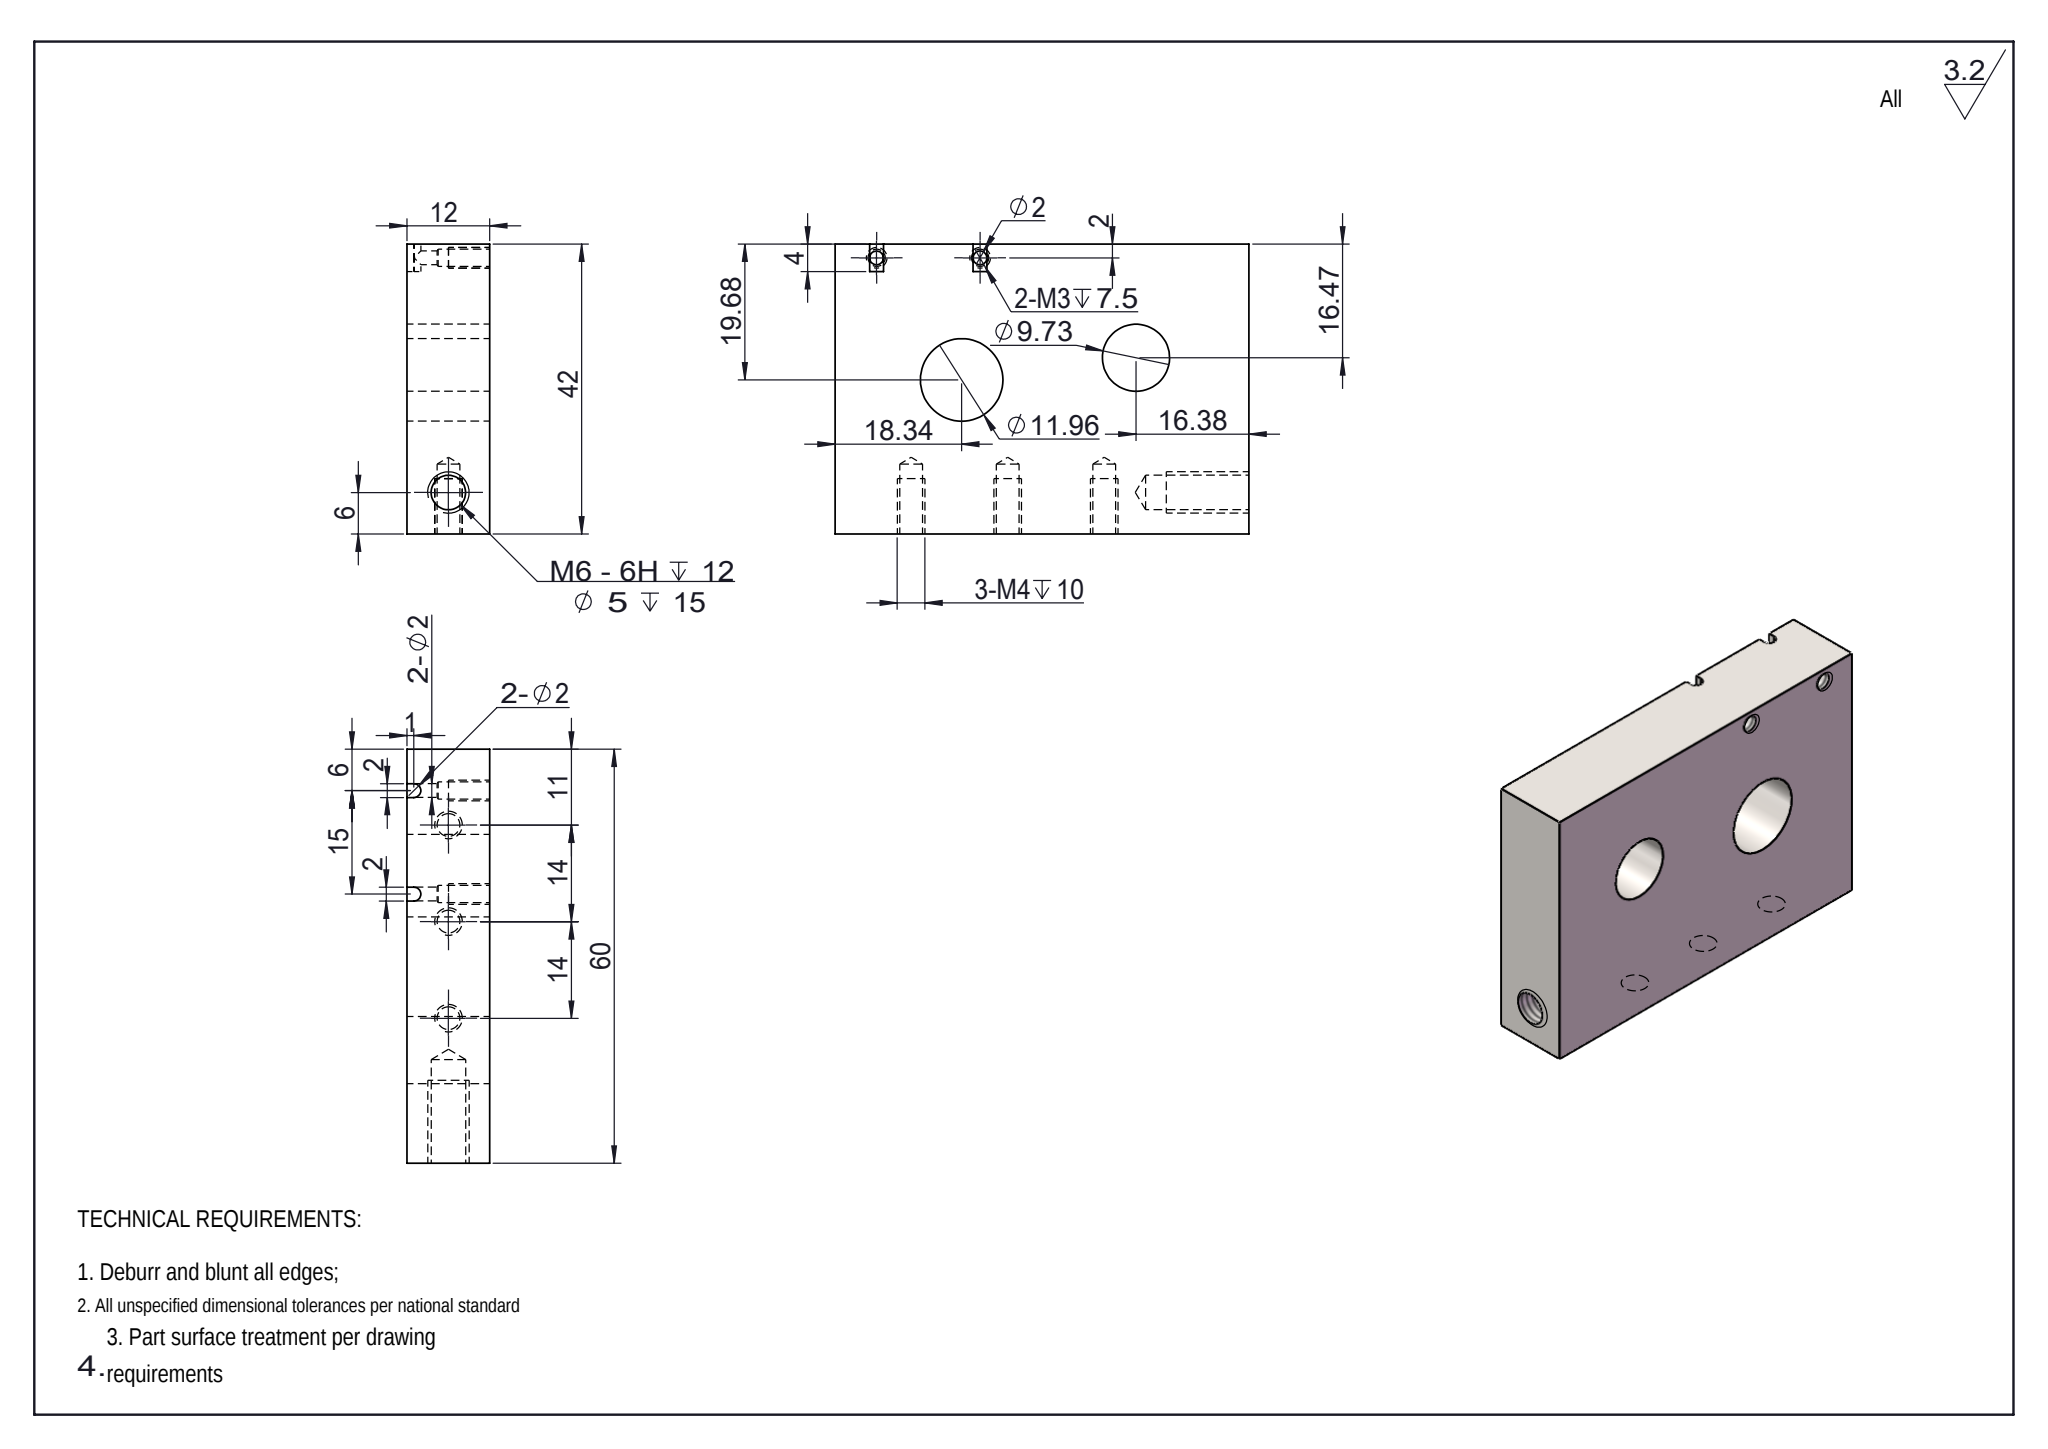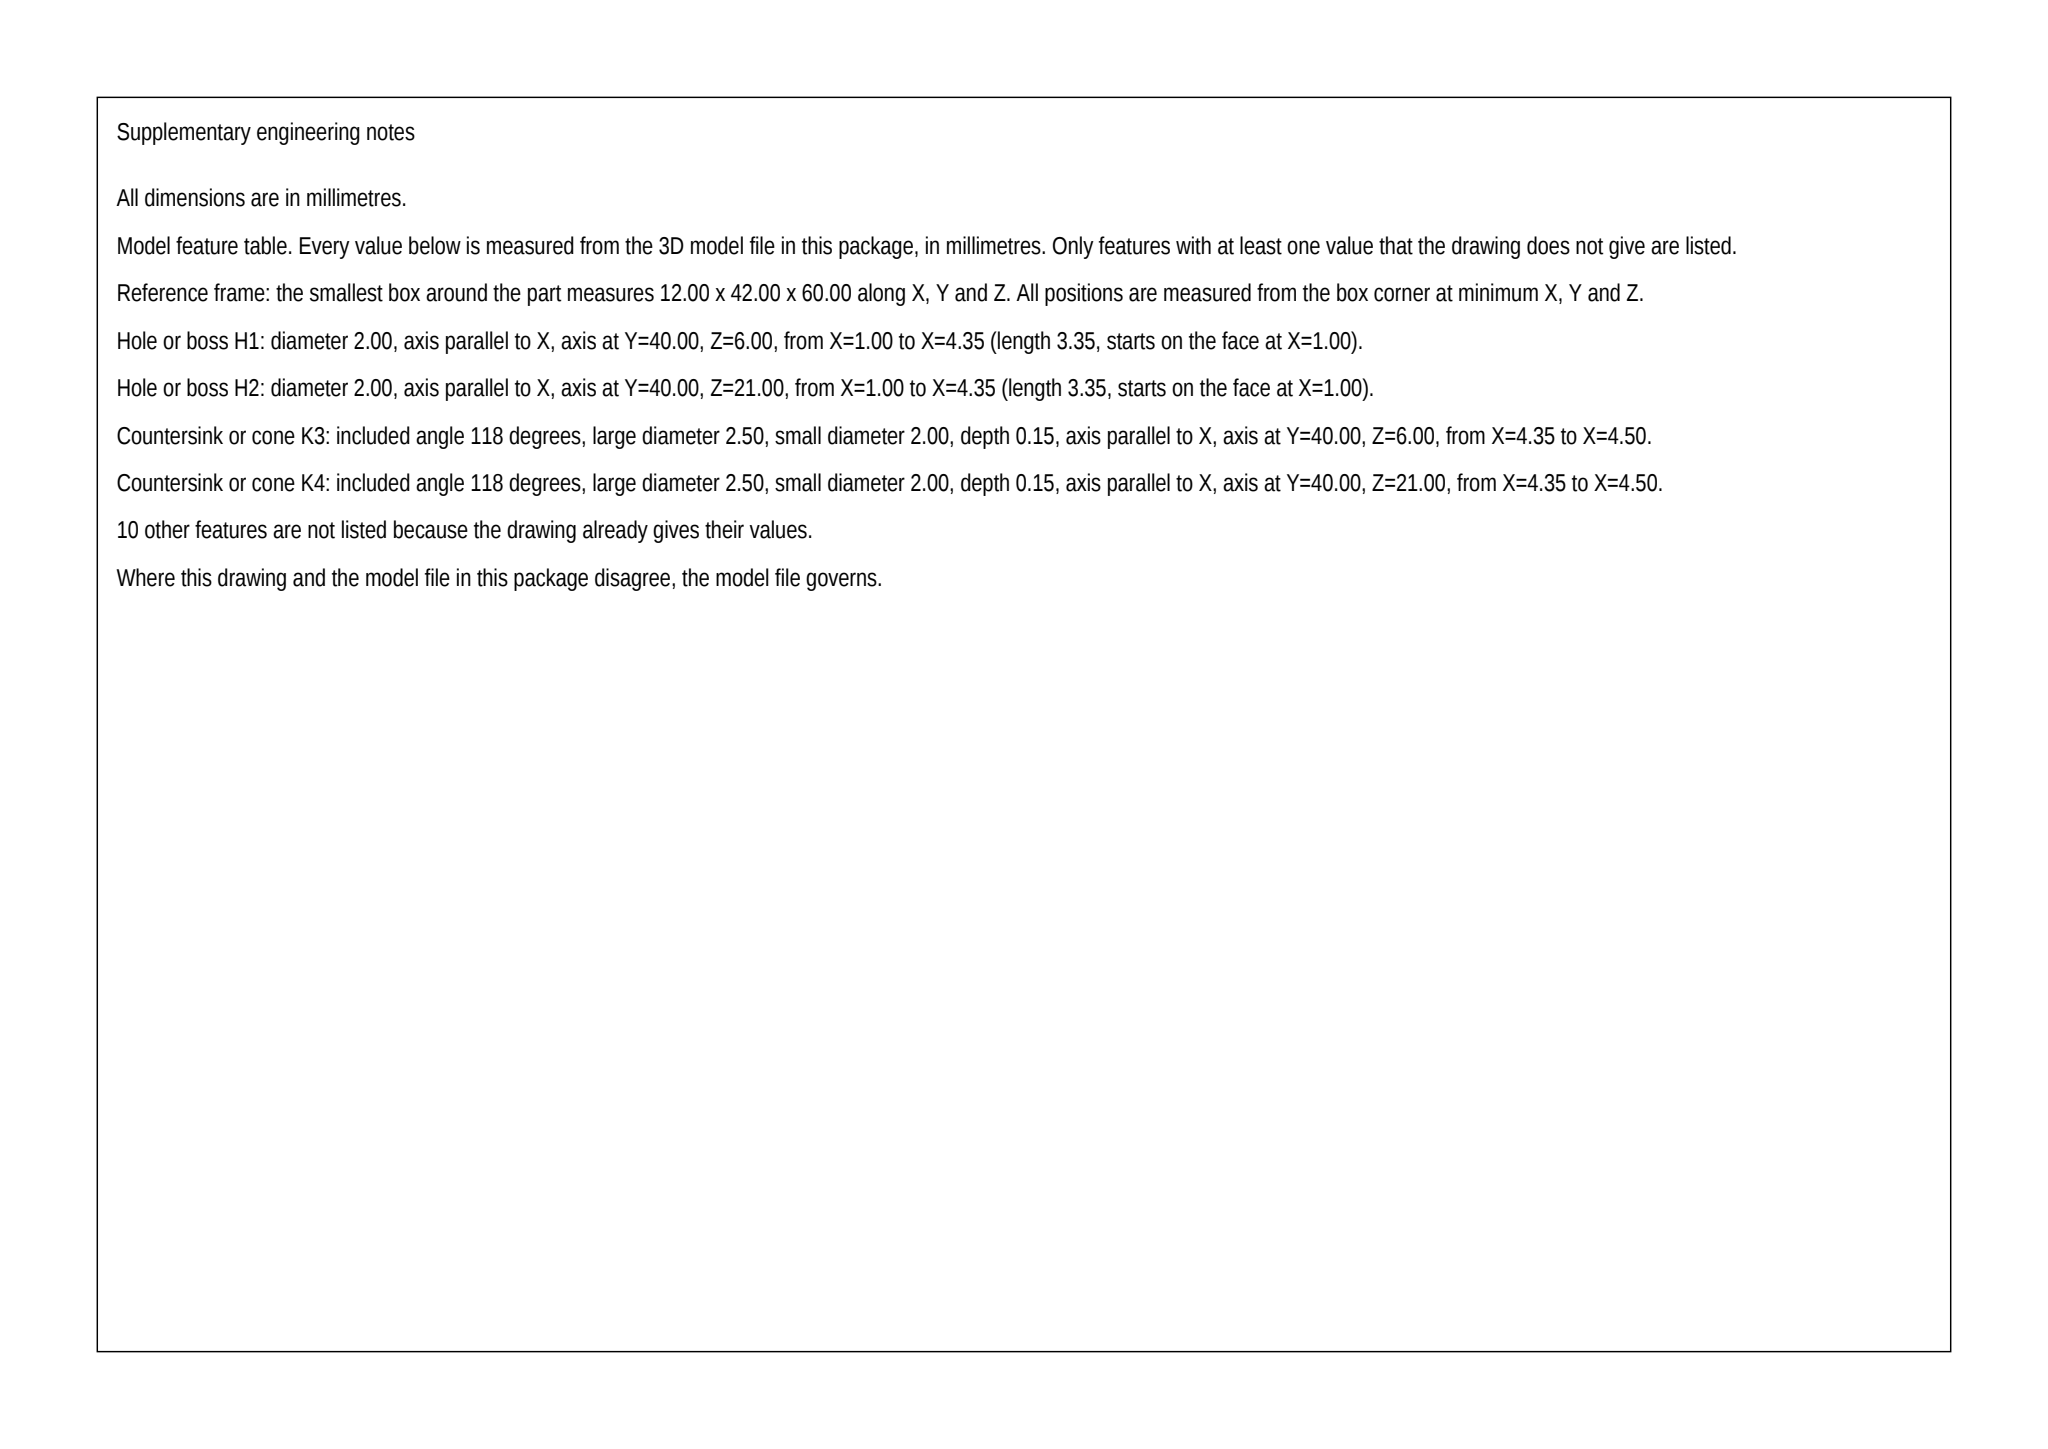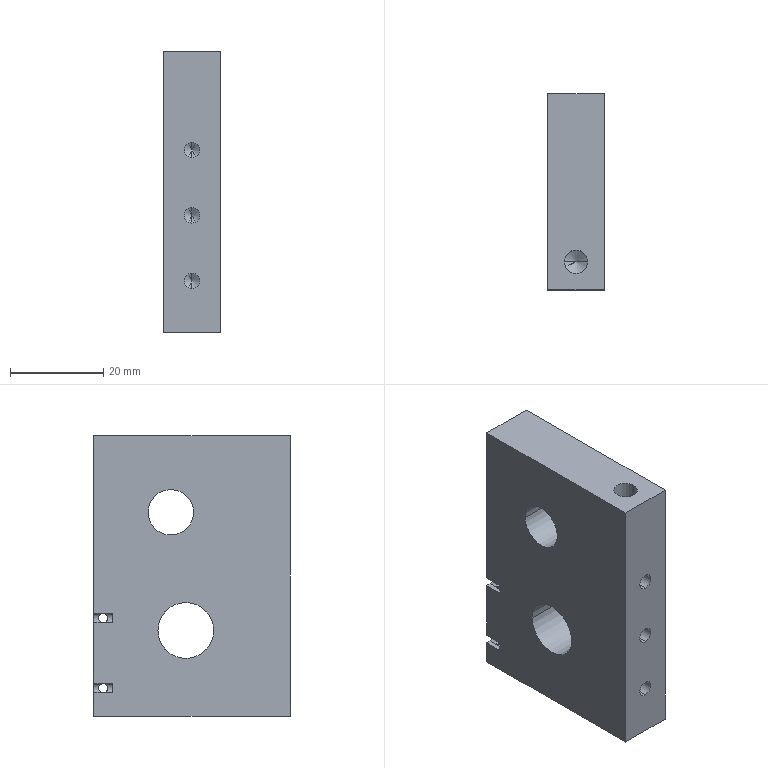Part | SolidWorks | mm | 1 solid | 48 faces | box 12 x 42 x 60 mm | volume 27308 mm3 | cylinder 24 | cone 12 | plane 12 | commonest cylinder face diameters 2 x8 3.3 x6 2.5 x4 9.734 x2 11.959 x2 5 x2
build123d program:
from build123d import *

# Parameters (mm, degrees)
SKETCH1_W             = 12
SKETCH1_H             = 42
BOSS_EXTRUDE1_DEPTH   = 60
CUT_EXTRUDE1_DEPTH    = 4
M3_TAPPED_HOLE1_D     = 2.5
M3_TAPPED_HOLE1_DEPTH = 7.5
M3_TAPPED_HOLE1_TIP   = 0.7511
SKETCH5_R             = 1
CUT_EXTRUDE2_DEPTH    = 75.216
M4_TAPPED_HOLE1_D     = 3.3
M4_TAPPED_HOLE1_DEPTH = 10.1
M4_TAPPED_HOLE1_TIP   = 0.9914
M6_TAPPED_HOLE1_D     = 5
M6_TAPPED_HOLE1_DEPTH = 15
M6_TAPPED_HOLE1_TIP   = 1.502
SKETCH10_R            = 4.867
SKETCH10_R_2          = 5.979
CUT_EXTRUDE3_DEPTH    = 850


with BuildPart() as part:
    # Sketch1 → Boss-Extrude1 (new body)
    with BuildSketch(Plane.XY):
        with Locations((6, 21)):
            Rectangle(SKETCH1_W, SKETCH1_H)
    extrude(amount=BOSS_EXTRUDE1_DEPTH)

    # Sketch2 → Cut-Extrude1 (cut)
    with BuildSketch(Plane(origin=(0, 42, 0), x_dir=(1, 0, 0), z_dir=(0, 1, 0))):
        with BuildLine():
            Line((1, -5), (0, -5))
            Line((0, -5), (0, -7))
            Line((0, -7), (1, -7))
            ThreePointArc((1, -7), (2, -6), (1, -5))
        make_face()
        with BuildLine():
            Line((1, -20), (0, -20))
            Line((0, -20), (0, -22))
            Line((0, -22), (1, -22))
            ThreePointArc((1, -22), (2, -21), (1, -20))
        make_face()
    extrude(amount=-CUT_EXTRUDE1_DEPTH, mode=Mode.SUBTRACT)

    # M3 Tapped Hole1
    with Locations(Plane(origin=(12, 0, 0), x_dir=(0, 0, -1), z_dir=(1, 0, 0))):
        with Locations((-6, 40), (-21, 40)):
            Hole(M3_TAPPED_HOLE1_D / 2, depth=M3_TAPPED_HOLE1_DEPTH)
            with Locations((0, 0, -(M3_TAPPED_HOLE1_DEPTH + M3_TAPPED_HOLE1_TIP / 2))):  # 118° drill point
                Cone(0, M3_TAPPED_HOLE1_D / 2, M3_TAPPED_HOLE1_TIP, mode=Mode.SUBTRACT)

    # Sketch5 → Cut-Extrude2 (cut, through all)
    with BuildSketch(Plane(origin=(12, 0, 0), x_dir=(0, 0, -1), z_dir=(1, 0, 0))):
        with Locations((-21, 40)):
            Circle(SKETCH5_R)
        with Locations((-6, 40)):
            Circle(SKETCH5_R)
    extrude(amount=-CUT_EXTRUDE2_DEPTH, mode=Mode.SUBTRACT)

    # M4 Tapped Hole1
    with Locations(Plane(origin=(0, 0, 0), x_dir=(-1, 0, 0), z_dir=(0, -1, 0))):
        with Locations((-6, -11), (-6, -25), (-6, -39)):
            Hole(M4_TAPPED_HOLE1_D / 2, depth=M4_TAPPED_HOLE1_DEPTH)
            with Locations((0, 0, -(M4_TAPPED_HOLE1_DEPTH + M4_TAPPED_HOLE1_TIP / 2))):  # 118° drill point
                Cone(0, M4_TAPPED_HOLE1_D / 2, M4_TAPPED_HOLE1_TIP, mode=Mode.SUBTRACT)

    # M6 Tapped Hole1
    with Locations(Plane.XY.offset(60)):
        with Locations((6, 6)):
            Hole(M6_TAPPED_HOLE1_D / 2, depth=M6_TAPPED_HOLE1_DEPTH)
            with Locations((0, 0, -(M6_TAPPED_HOLE1_DEPTH + M6_TAPPED_HOLE1_TIP / 2))):  # 118° drill point
                Cone(0, M6_TAPPED_HOLE1_D / 2, M6_TAPPED_HOLE1_TIP, mode=Mode.SUBTRACT)

    # Sketch10 → Cut-Extrude3 (cut)
    with BuildSketch(Plane.ZY):
        with Locations(Location((43.622, 25.53, 0), (0, 0, 270))):
            Circle(SKETCH10_R)
        with Locations(Location((18.341, 22.315, 0), (0, 0, 270))):
            Circle(SKETCH10_R_2)
    extrude(amount=-CUT_EXTRUDE3_DEPTH, mode=Mode.SUBTRACT)


solid = part.part